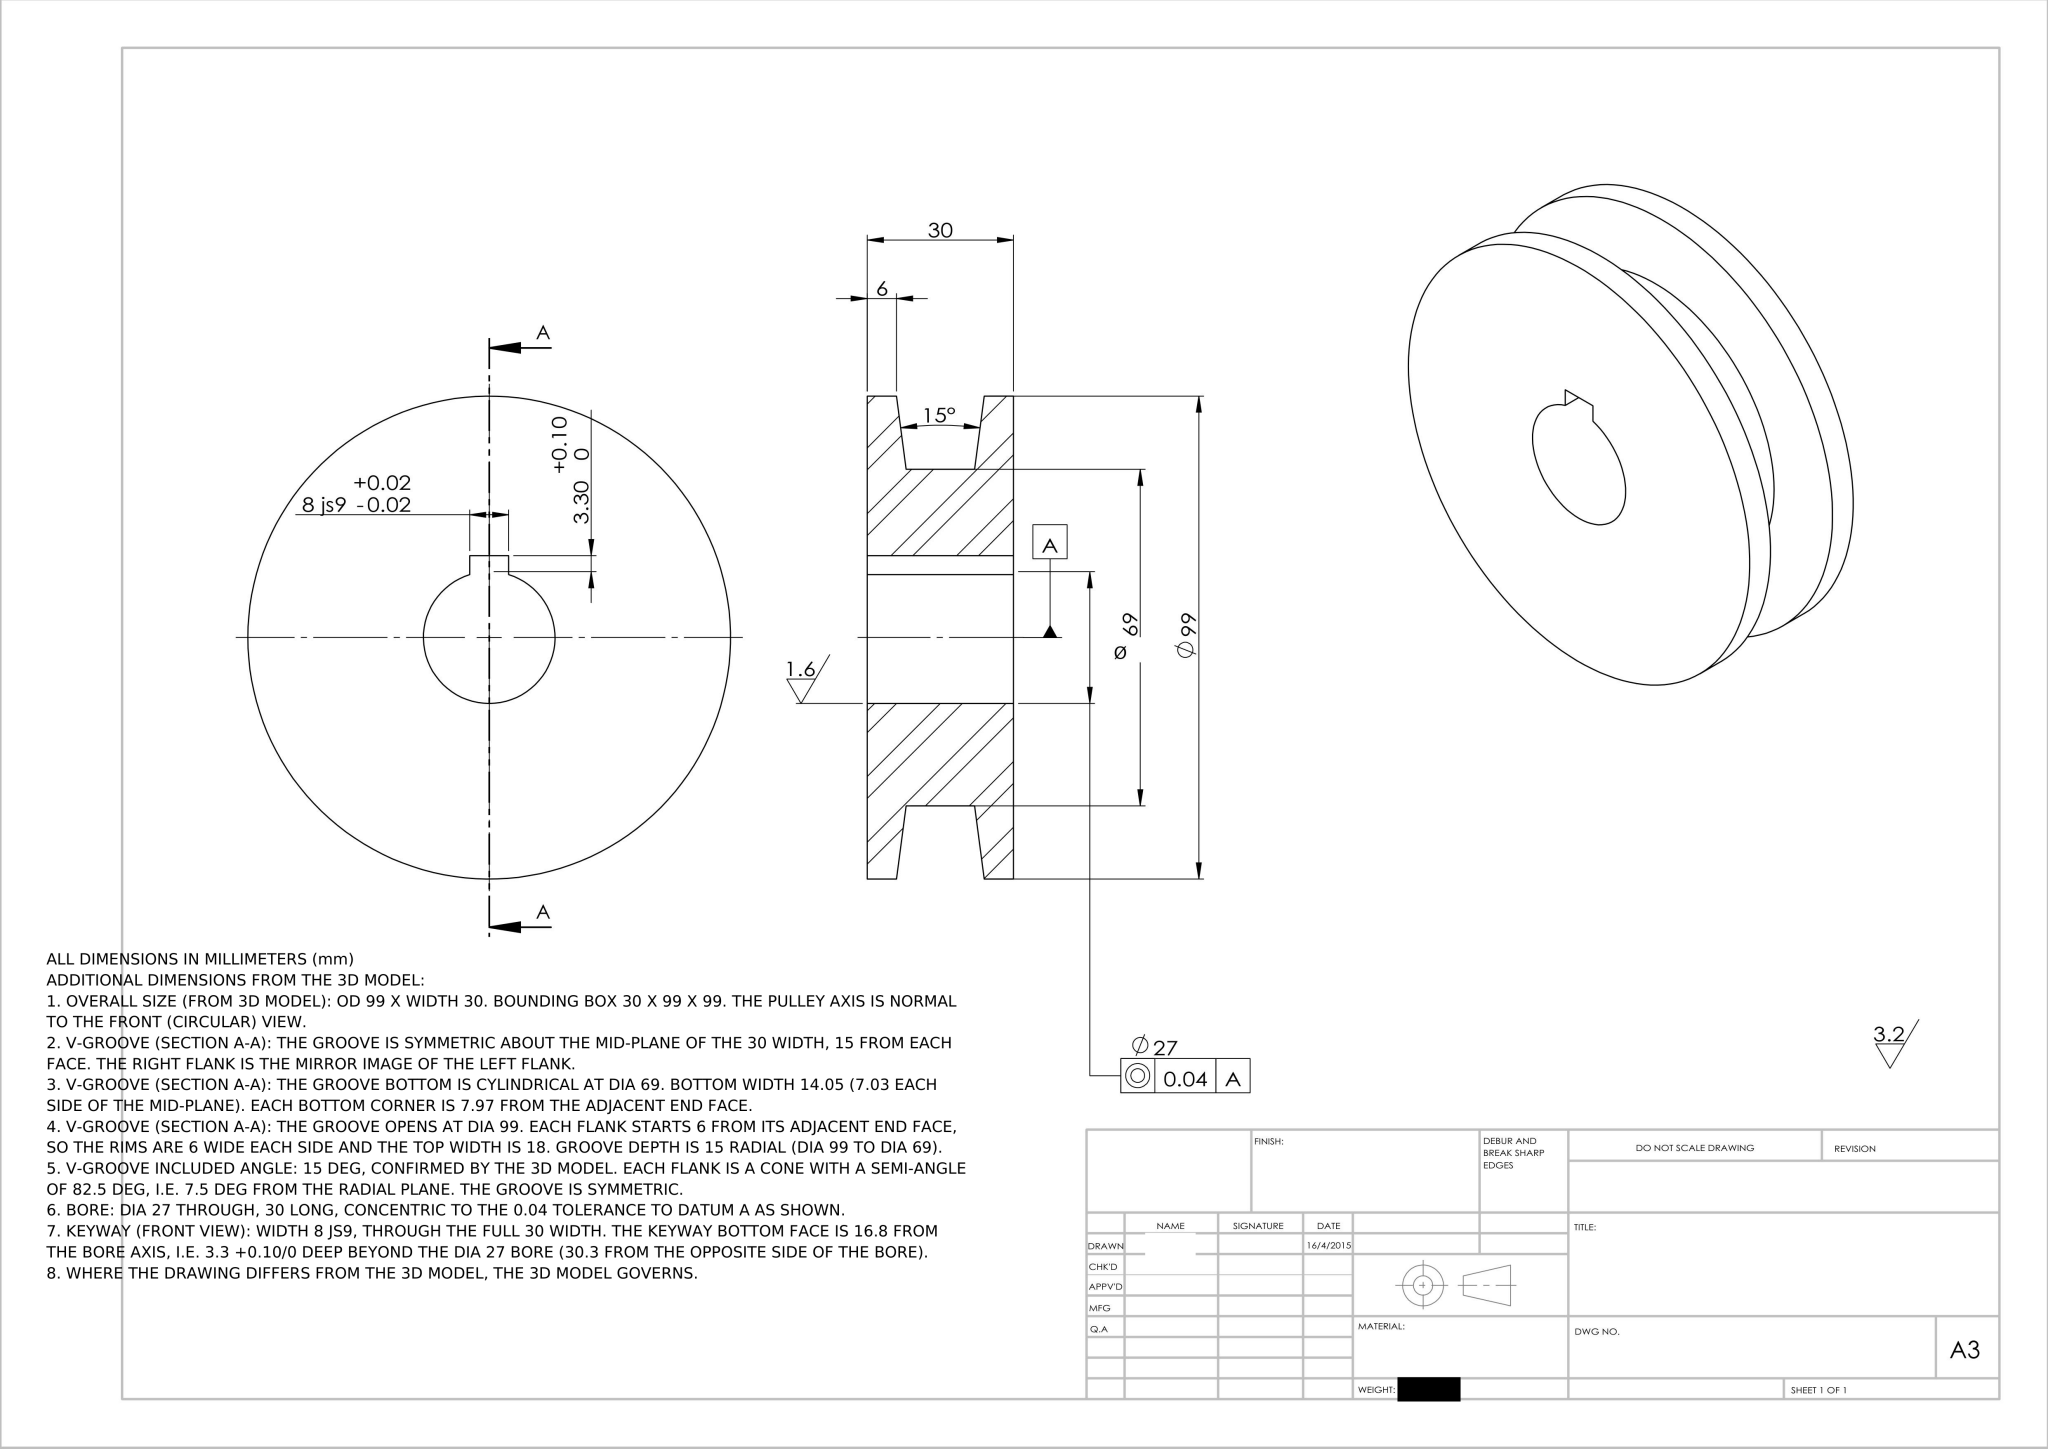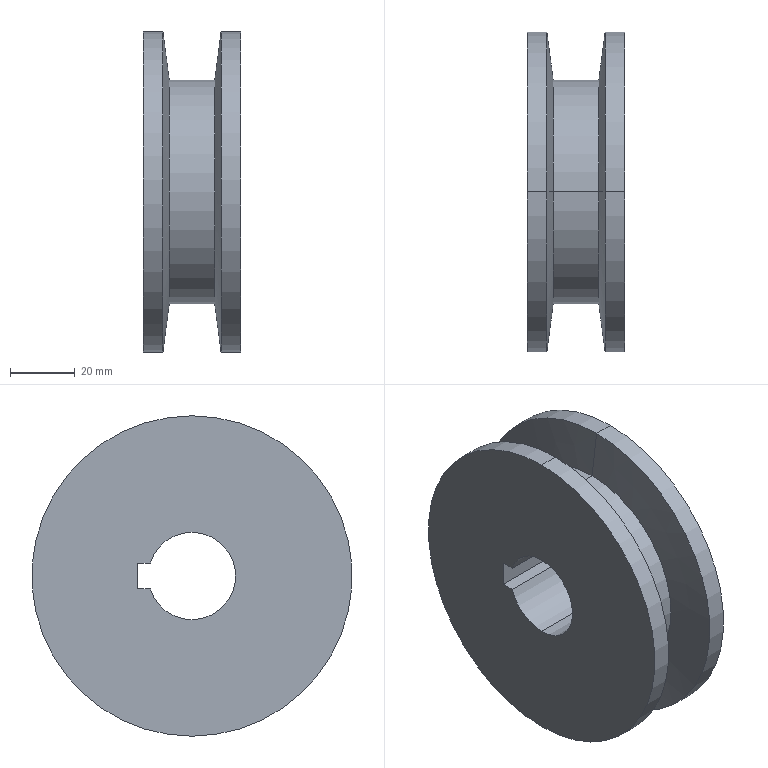Part | NX | mm | Keyed Bore Flanged Pulley | 1 solid | 18 faces | box 30 x 99 x 99 mm | volume 149014 mm3 | cylinder 9 | plane 5 | cone 4 | commonest cylinder face diameters 99 x4 27 x3 69 x2
STEP:
#1=COLOUR_RGB('',0.7922,0.8196,0.9333);
#2=FILL_AREA_STYLE_COLOUR('',#1);
#3=FILL_AREA_STYLE('',(#2));
#4=SURFACE_STYLE_FILL_AREA(#3);
#5=SURFACE_SIDE_STYLE('',(#4));
#6=SURFACE_STYLE_USAGE(.BOTH.,#5);
#7=PRESENTATION_STYLE_ASSIGNMENT((#6));
#8=CARTESIAN_POINT('',(15.,0.,49.5));
#9=VERTEX_POINT('',#8);
#10=CARTESIAN_POINT('',(15.,0.,-49.5));
#11=VERTEX_POINT('',#10);
#12=CARTESIAN_POINT('',(15.,0.,0.));
#13=DIRECTION('',(-1.,0.,0.));
#14=DIRECTION('',(0.,0.,1.));
#15=AXIS2_PLACEMENT_3D('',#12,#13,#14);
#16=CIRCLE('',#15,49.5);
#17=EDGE_CURVE('',#9,#11,#16,.T.);
#18=ORIENTED_EDGE('',*,*,#17,.T.);
#19=CARTESIAN_POINT('',(9.,0.,-49.5));
#20=VERTEX_POINT('',#19);
#21=CARTESIAN_POINT('',(0.,0.,-49.5));
#22=DIRECTION('',(-1.,0.,0.));
#23=VECTOR('',#22,1000.);
#24=LINE('',#21,#23);
#25=EDGE_CURVE('',#11,#20,#24,.T.);
#26=ORIENTED_EDGE('',*,*,#25,.T.);
#27=CARTESIAN_POINT('',(9.,0.,49.5));
#28=VERTEX_POINT('',#27);
#29=CARTESIAN_POINT('',(9.,0.,0.));
#30=DIRECTION('',(-1.,0.,0.));
#31=DIRECTION('',(0.,0.,1.));
#32=AXIS2_PLACEMENT_3D('',#29,#30,#31);
#33=CIRCLE('',#32,49.5);
#34=EDGE_CURVE('',#28,#20,#33,.T.);
#35=ORIENTED_EDGE('',*,*,#34,.F.);
#36=CARTESIAN_POINT('',(0.,0.,49.5));
#37=DIRECTION('',(-1.,0.,0.));
#38=VECTOR('',#37,1000.);
#39=LINE('',#36,#38);
#40=EDGE_CURVE('',#9,#28,#39,.T.);
#41=ORIENTED_EDGE('',*,*,#40,.F.);
#42=EDGE_LOOP('',(#18,#26,#35,#41));
#43=FACE_OUTER_BOUND('',#42,.T.);
#44=CARTESIAN_POINT('',(0.,0.,0.));
#45=DIRECTION('',(-1.,0.,0.));
#46=DIRECTION('',(0.,0.,1.));
#47=AXIS2_PLACEMENT_3D('',#44,#45,#46);
#48=CYLINDRICAL_SURFACE('',#47,49.5);
#49=ADVANCED_FACE('',(#43),#48,.T.);
#50=CARTESIAN_POINT('',(7.025,0.,34.5));
#51=VERTEX_POINT('',#50);
#52=CARTESIAN_POINT('',(7.025,0.,-34.5));
#53=VERTEX_POINT('',#52);
#54=CARTESIAN_POINT('',(7.025,0.,0.));
#55=DIRECTION('',(-1.,0.,0.));
#56=DIRECTION('',(0.,0.,1.));
#57=AXIS2_PLACEMENT_3D('',#54,#55,#56);
#58=CIRCLE('',#57,34.5);
#59=EDGE_CURVE('',#51,#53,#58,.T.);
#60=ORIENTED_EDGE('',*,*,#59,.F.);
#61=CARTESIAN_POINT('',(9.,0.,49.5));
#62=DIRECTION('',(0.1305,0.,0.9914));
#63=VECTOR('',#62,1000.);
#64=LINE('',#61,#63);
#65=EDGE_CURVE('',#51,#28,#64,.T.);
#66=ORIENTED_EDGE('',*,*,#65,.T.);
#67=ORIENTED_EDGE('',*,*,#34,.T.);
#68=CARTESIAN_POINT('',(9.,0.,-49.5));
#69=DIRECTION('',(0.1305,0.,-0.9914));
#70=VECTOR('',#69,1000.);
#71=LINE('',#68,#70);
#72=EDGE_CURVE('',#53,#20,#71,.T.);
#73=ORIENTED_EDGE('',*,*,#72,.F.);
#74=EDGE_LOOP('',(#60,#66,#67,#73));
#75=FACE_OUTER_BOUND('',#74,.T.);
#76=CARTESIAN_POINT('',(9.,0.,0.));
#77=DIRECTION('',(1.,0.,0.));
#78=DIRECTION('',(0.,0.,-1.));
#79=AXIS2_PLACEMENT_3D('',#76,#77,#78);
#80=CONICAL_SURFACE('',#79,49.5,1.44);
#81=ADVANCED_FACE('',(#75),#80,.T.);
#82=ORIENTED_EDGE('',*,*,#59,.T.);
#83=CARTESIAN_POINT('',(-7.025,0.,-34.5));
#84=VERTEX_POINT('',#83);
#85=CARTESIAN_POINT('',(0.,0.,-34.5));
#86=DIRECTION('',(-1.,0.,0.));
#87=VECTOR('',#86,1000.);
#88=LINE('',#85,#87);
#89=EDGE_CURVE('',#53,#84,#88,.T.);
#90=ORIENTED_EDGE('',*,*,#89,.T.);
#91=CARTESIAN_POINT('',(-7.025,0.,34.5));
#92=VERTEX_POINT('',#91);
#93=CARTESIAN_POINT('',(-7.025,0.,0.));
#94=DIRECTION('',(-1.,0.,0.));
#95=DIRECTION('',(0.,0.,1.));
#96=AXIS2_PLACEMENT_3D('',#93,#94,#95);
#97=CIRCLE('',#96,34.5);
#98=EDGE_CURVE('',#92,#84,#97,.T.);
#99=ORIENTED_EDGE('',*,*,#98,.F.);
#100=CARTESIAN_POINT('',(0.,0.,34.5));
#101=DIRECTION('',(-1.,0.,0.));
#102=VECTOR('',#101,1000.);
#103=LINE('',#100,#102);
#104=EDGE_CURVE('',#51,#92,#103,.T.);
#105=ORIENTED_EDGE('',*,*,#104,.F.);
#106=EDGE_LOOP('',(#82,#90,#99,#105));
#107=FACE_OUTER_BOUND('',#106,.T.);
#108=CARTESIAN_POINT('',(0.,0.,0.));
#109=DIRECTION('',(-1.,0.,0.));
#110=DIRECTION('',(0.,0.,1.));
#111=AXIS2_PLACEMENT_3D('',#108,#109,#110);
#112=CYLINDRICAL_SURFACE('',#111,34.5);
#113=ADVANCED_FACE('',(#107),#112,.T.);
#114=ORIENTED_EDGE('',*,*,#98,.T.);
#115=CARTESIAN_POINT('',(-9.,0.,-49.5));
#116=VERTEX_POINT('',#115);
#117=CARTESIAN_POINT('',(-7.025,0.,-34.5));
#118=DIRECTION('',(-0.1305,0.,-0.9914));
#119=VECTOR('',#118,1000.);
#120=LINE('',#117,#119);
#121=EDGE_CURVE('',#84,#116,#120,.T.);
#122=ORIENTED_EDGE('',*,*,#121,.T.);
#123=CARTESIAN_POINT('',(-9.,0.,49.5));
#124=VERTEX_POINT('',#123);
#125=CARTESIAN_POINT('',(-9.,0.,0.));
#126=DIRECTION('',(-1.,0.,0.));
#127=DIRECTION('',(0.,0.,1.));
#128=AXIS2_PLACEMENT_3D('',#125,#126,#127);
#129=CIRCLE('',#128,49.5);
#130=EDGE_CURVE('',#124,#116,#129,.T.);
#131=ORIENTED_EDGE('',*,*,#130,.F.);
#132=CARTESIAN_POINT('',(-7.025,0.,34.5));
#133=DIRECTION('',(-0.1305,0.,0.9914));
#134=VECTOR('',#133,1000.);
#135=LINE('',#132,#134);
#136=EDGE_CURVE('',#92,#124,#135,.T.);
#137=ORIENTED_EDGE('',*,*,#136,.F.);
#138=EDGE_LOOP('',(#114,#122,#131,#137));
#139=FACE_OUTER_BOUND('',#138,.T.);
#140=CARTESIAN_POINT('',(-7.025,0.,0.));
#141=DIRECTION('',(-1.,0.,0.));
#142=DIRECTION('',(0.,0.,1.));
#143=AXIS2_PLACEMENT_3D('',#140,#141,#142);
#144=CONICAL_SURFACE('',#143,34.5,1.44);
#145=ADVANCED_FACE('',(#139),#144,.T.);
#146=ORIENTED_EDGE('',*,*,#130,.T.);
#147=CARTESIAN_POINT('',(-15.,0.,-49.5));
#148=VERTEX_POINT('',#147);
#149=CARTESIAN_POINT('',(0.,0.,-49.5));
#150=DIRECTION('',(-1.,0.,0.));
#151=VECTOR('',#150,1000.);
#152=LINE('',#149,#151);
#153=EDGE_CURVE('',#116,#148,#152,.T.);
#154=ORIENTED_EDGE('',*,*,#153,.T.);
#155=CARTESIAN_POINT('',(-15.,0.,49.5));
#156=VERTEX_POINT('',#155);
#157=CARTESIAN_POINT('',(-15.,0.,0.));
#158=DIRECTION('',(-1.,0.,0.));
#159=DIRECTION('',(0.,0.,1.));
#160=AXIS2_PLACEMENT_3D('',#157,#158,#159);
#161=CIRCLE('',#160,49.5);
#162=EDGE_CURVE('',#156,#148,#161,.T.);
#163=ORIENTED_EDGE('',*,*,#162,.F.);
#164=CARTESIAN_POINT('',(0.,0.,49.5));
#165=DIRECTION('',(-1.,0.,0.));
#166=VECTOR('',#165,1000.);
#167=LINE('',#164,#166);
#168=EDGE_CURVE('',#124,#156,#167,.T.);
#169=ORIENTED_EDGE('',*,*,#168,.F.);
#170=EDGE_LOOP('',(#146,#154,#163,#169));
#171=FACE_OUTER_BOUND('',#170,.T.);
#172=CARTESIAN_POINT('',(0.,0.,0.));
#173=DIRECTION('',(-1.,0.,0.));
#174=DIRECTION('',(0.,0.,1.));
#175=AXIS2_PLACEMENT_3D('',#172,#173,#174);
#176=CYLINDRICAL_SURFACE('',#175,49.5);
#177=ADVANCED_FACE('',(#171),#176,.T.);
#178=CARTESIAN_POINT('',(15.,0.,-13.5));
#179=VERTEX_POINT('',#178);
#180=CARTESIAN_POINT('',(15.,0.,13.5));
#181=VERTEX_POINT('',#180);
#182=CARTESIAN_POINT('',(15.,0.,0.));
#183=DIRECTION('',(-1.,0.,0.));
#184=DIRECTION('',(0.,0.,1.));
#185=AXIS2_PLACEMENT_3D('',#182,#183,#184);
#186=CIRCLE('',#185,13.5);
#187=EDGE_CURVE('',#179,#181,#186,.T.);
#188=ORIENTED_EDGE('',*,*,#187,.F.);
#189=CARTESIAN_POINT('',(-15.,0.,-13.5));
#190=VERTEX_POINT('',#189);
#191=CARTESIAN_POINT('',(0.,0.,-13.5));
#192=DIRECTION('',(-1.,0.,0.));
#193=VECTOR('',#192,1000.);
#194=LINE('',#191,#193);
#195=EDGE_CURVE('',#179,#190,#194,.T.);
#196=ORIENTED_EDGE('',*,*,#195,.T.);
#197=CARTESIAN_POINT('',(-15.,0.,13.5));
#198=VERTEX_POINT('',#197);
#199=CARTESIAN_POINT('',(-15.,0.,0.));
#200=DIRECTION('',(-1.,0.,0.));
#201=DIRECTION('',(0.,0.,1.));
#202=AXIS2_PLACEMENT_3D('',#199,#200,#201);
#203=CIRCLE('',#202,13.5);
#204=EDGE_CURVE('',#190,#198,#203,.T.);
#205=ORIENTED_EDGE('',*,*,#204,.T.);
#206=CARTESIAN_POINT('',(0.,0.,13.5));
#207=DIRECTION('',(-1.,0.,0.));
#208=VECTOR('',#207,1000.);
#209=LINE('',#206,#208);
#210=EDGE_CURVE('',#181,#198,#209,.T.);
#211=ORIENTED_EDGE('',*,*,#210,.F.);
#212=EDGE_LOOP('',(#188,#196,#205,#211));
#213=FACE_OUTER_BOUND('',#212,.T.);
#214=CARTESIAN_POINT('',(0.,0.,0.));
#215=DIRECTION('',(-1.,0.,0.));
#216=DIRECTION('',(0.,0.,1.));
#217=AXIS2_PLACEMENT_3D('',#214,#215,#216);
#218=CYLINDRICAL_SURFACE('',#217,13.5);
#219=ADVANCED_FACE('',(#213),#218,.F.);
#220=CARTESIAN_POINT('',(15.,12.894,4.));
#221=VERTEX_POINT('',#220);
#222=CARTESIAN_POINT('',(15.,0.,0.));
#223=DIRECTION('',(-1.,0.,0.));
#224=DIRECTION('',(0.,0.,1.));
#225=AXIS2_PLACEMENT_3D('',#222,#223,#224);
#226=CIRCLE('',#225,13.5);
#227=EDGE_CURVE('',#181,#221,#226,.T.);
#228=ORIENTED_EDGE('',*,*,#227,.F.);
#229=ORIENTED_EDGE('',*,*,#210,.T.);
#230=CARTESIAN_POINT('',(-15.,12.894,4.));
#231=VERTEX_POINT('',#230);
#232=CARTESIAN_POINT('',(-15.,0.,0.));
#233=DIRECTION('',(-1.,0.,0.));
#234=DIRECTION('',(0.,0.,1.));
#235=AXIS2_PLACEMENT_3D('',#232,#233,#234);
#236=CIRCLE('',#235,13.5);
#237=EDGE_CURVE('',#198,#231,#236,.T.);
#238=ORIENTED_EDGE('',*,*,#237,.T.);
#239=CARTESIAN_POINT('',(-15.,12.894,4.));
#240=DIRECTION('',(1.,0.,0.));
#241=VECTOR('',#240,1000.);
#242=LINE('',#239,#241);
#243=EDGE_CURVE('',#231,#221,#242,.T.);
#244=ORIENTED_EDGE('',*,*,#243,.T.);
#245=EDGE_LOOP('',(#228,#229,#238,#244));
#246=FACE_OUTER_BOUND('',#245,.T.);
#247=CARTESIAN_POINT('',(0.,0.,0.));
#248=DIRECTION('',(-1.,0.,0.));
#249=DIRECTION('',(0.,0.,1.));
#250=AXIS2_PLACEMENT_3D('',#247,#248,#249);
#251=CYLINDRICAL_SURFACE('',#250,13.5);
#252=ADVANCED_FACE('',(#246),#251,.F.);
#253=ORIENTED_EDGE('',*,*,#195,.F.);
#254=CARTESIAN_POINT('',(15.,12.894,-4.));
#255=VERTEX_POINT('',#254);
#256=CARTESIAN_POINT('',(15.,0.,0.));
#257=DIRECTION('',(-1.,0.,0.));
#258=DIRECTION('',(0.,0.,1.));
#259=AXIS2_PLACEMENT_3D('',#256,#257,#258);
#260=CIRCLE('',#259,13.5);
#261=EDGE_CURVE('',#255,#179,#260,.T.);
#262=ORIENTED_EDGE('',*,*,#261,.F.);
#263=CARTESIAN_POINT('',(-15.,12.894,-4.));
#264=VERTEX_POINT('',#263);
#265=CARTESIAN_POINT('',(-15.,12.894,-4.));
#266=DIRECTION('',(1.,0.,0.));
#267=VECTOR('',#266,1000.);
#268=LINE('',#265,#267);
#269=EDGE_CURVE('',#264,#255,#268,.T.);
#270=ORIENTED_EDGE('',*,*,#269,.F.);
#271=CARTESIAN_POINT('',(-15.,0.,0.));
#272=DIRECTION('',(-1.,0.,0.));
#273=DIRECTION('',(0.,0.,1.));
#274=AXIS2_PLACEMENT_3D('',#271,#272,#273);
#275=CIRCLE('',#274,13.5);
#276=EDGE_CURVE('',#264,#190,#275,.T.);
#277=ORIENTED_EDGE('',*,*,#276,.T.);
#278=EDGE_LOOP('',(#253,#262,#270,#277));
#279=FACE_OUTER_BOUND('',#278,.T.);
#280=CARTESIAN_POINT('',(0.,0.,0.));
#281=DIRECTION('',(-1.,0.,0.));
#282=DIRECTION('',(0.,0.,1.));
#283=AXIS2_PLACEMENT_3D('',#280,#281,#282);
#284=CYLINDRICAL_SURFACE('',#283,13.5);
#285=ADVANCED_FACE('',(#279),#284,.F.);
#286=CARTESIAN_POINT('',(-15.,16.8,-4.));
#287=VERTEX_POINT('',#286);
#288=CARTESIAN_POINT('',(-15.,16.8,4.));
#289=VERTEX_POINT('',#288);
#290=CARTESIAN_POINT('',(-15.,16.8,4.));
#291=DIRECTION('',(0.,0.,1.));
#292=VECTOR('',#291,1000.);
#293=LINE('',#290,#292);
#294=EDGE_CURVE('',#287,#289,#293,.T.);
#295=ORIENTED_EDGE('',*,*,#294,.T.);
#296=CARTESIAN_POINT('',(-15.,12.894,4.));
#297=DIRECTION('',(0.,-1.,0.));
#298=VECTOR('',#297,1000.);
#299=LINE('',#296,#298);
#300=EDGE_CURVE('',#289,#231,#299,.T.);
#301=ORIENTED_EDGE('',*,*,#300,.T.);
#302=ORIENTED_EDGE('',*,*,#237,.F.);
#303=ORIENTED_EDGE('',*,*,#204,.F.);
#304=ORIENTED_EDGE('',*,*,#276,.F.);
#305=CARTESIAN_POINT('',(-15.,16.8,-4.));
#306=DIRECTION('',(0.,1.,0.));
#307=VECTOR('',#306,1000.);
#308=LINE('',#305,#307);
#309=EDGE_CURVE('',#264,#287,#308,.T.);
#310=ORIENTED_EDGE('',*,*,#309,.T.);
#311=EDGE_LOOP('',(#295,#301,#302,#303,#304,#310));
#312=FACE_BOUND('',#311,.T.);
#313=ORIENTED_EDGE('',*,*,#162,.T.);
#314=CARTESIAN_POINT('',(-15.,0.,0.));
#315=DIRECTION('',(-1.,0.,0.));
#316=DIRECTION('',(0.,0.,1.));
#317=AXIS2_PLACEMENT_3D('',#314,#315,#316);
#318=CIRCLE('',#317,49.5);
#319=EDGE_CURVE('',#148,#156,#318,.T.);
#320=ORIENTED_EDGE('',*,*,#319,.T.);
#321=EDGE_LOOP('',(#313,#320));
#322=FACE_OUTER_BOUND('',#321,.T.);
#323=CARTESIAN_POINT('',(-15.,13.5,0.));
#324=DIRECTION('',(1.,0.,0.));
#325=DIRECTION('',(0.,0.,-1.));
#326=AXIS2_PLACEMENT_3D('',#323,#324,#325);
#327=PLANE('',#326);
#328=ADVANCED_FACE('',(#312,#322),#327,.F.);
#329=ORIENTED_EDGE('',*,*,#153,.F.);
#330=CARTESIAN_POINT('',(-9.,0.,0.));
#331=DIRECTION('',(-1.,0.,0.));
#332=DIRECTION('',(0.,0.,1.));
#333=AXIS2_PLACEMENT_3D('',#330,#331,#332);
#334=CIRCLE('',#333,49.5);
#335=EDGE_CURVE('',#116,#124,#334,.T.);
#336=ORIENTED_EDGE('',*,*,#335,.T.);
#337=ORIENTED_EDGE('',*,*,#168,.T.);
#338=ORIENTED_EDGE('',*,*,#319,.F.);
#339=EDGE_LOOP('',(#329,#336,#337,#338));
#340=FACE_OUTER_BOUND('',#339,.T.);
#341=CARTESIAN_POINT('',(0.,0.,0.));
#342=DIRECTION('',(-1.,0.,0.));
#343=DIRECTION('',(0.,0.,1.));
#344=AXIS2_PLACEMENT_3D('',#341,#342,#343);
#345=CYLINDRICAL_SURFACE('',#344,49.5);
#346=ADVANCED_FACE('',(#340),#345,.T.);
#347=ORIENTED_EDGE('',*,*,#121,.F.);
#348=CARTESIAN_POINT('',(-7.025,0.,0.));
#349=DIRECTION('',(-1.,0.,0.));
#350=DIRECTION('',(0.,0.,1.));
#351=AXIS2_PLACEMENT_3D('',#348,#349,#350);
#352=CIRCLE('',#351,34.5);
#353=EDGE_CURVE('',#84,#92,#352,.T.);
#354=ORIENTED_EDGE('',*,*,#353,.T.);
#355=ORIENTED_EDGE('',*,*,#136,.T.);
#356=ORIENTED_EDGE('',*,*,#335,.F.);
#357=EDGE_LOOP('',(#347,#354,#355,#356));
#358=FACE_OUTER_BOUND('',#357,.T.);
#359=CARTESIAN_POINT('',(-7.025,0.,0.));
#360=DIRECTION('',(-1.,0.,0.));
#361=DIRECTION('',(0.,0.,1.));
#362=AXIS2_PLACEMENT_3D('',#359,#360,#361);
#363=CONICAL_SURFACE('',#362,34.5,1.44);
#364=ADVANCED_FACE('',(#358),#363,.T.);
#365=ORIENTED_EDGE('',*,*,#89,.F.);
#366=CARTESIAN_POINT('',(7.025,0.,0.));
#367=DIRECTION('',(-1.,0.,0.));
#368=DIRECTION('',(0.,0.,1.));
#369=AXIS2_PLACEMENT_3D('',#366,#367,#368);
#370=CIRCLE('',#369,34.5);
#371=EDGE_CURVE('',#53,#51,#370,.T.);
#372=ORIENTED_EDGE('',*,*,#371,.T.);
#373=ORIENTED_EDGE('',*,*,#104,.T.);
#374=ORIENTED_EDGE('',*,*,#353,.F.);
#375=EDGE_LOOP('',(#365,#372,#373,#374));
#376=FACE_OUTER_BOUND('',#375,.T.);
#377=CARTESIAN_POINT('',(0.,0.,0.));
#378=DIRECTION('',(-1.,0.,0.));
#379=DIRECTION('',(0.,0.,1.));
#380=AXIS2_PLACEMENT_3D('',#377,#378,#379);
#381=CYLINDRICAL_SURFACE('',#380,34.5);
#382=ADVANCED_FACE('',(#376),#381,.T.);
#383=ORIENTED_EDGE('',*,*,#65,.F.);
#384=ORIENTED_EDGE('',*,*,#371,.F.);
#385=ORIENTED_EDGE('',*,*,#72,.T.);
#386=CARTESIAN_POINT('',(9.,0.,0.));
#387=DIRECTION('',(-1.,0.,0.));
#388=DIRECTION('',(0.,0.,1.));
#389=AXIS2_PLACEMENT_3D('',#386,#387,#388);
#390=CIRCLE('',#389,49.5);
#391=EDGE_CURVE('',#20,#28,#390,.T.);
#392=ORIENTED_EDGE('',*,*,#391,.T.);
#393=EDGE_LOOP('',(#383,#384,#385,#392));
#394=FACE_OUTER_BOUND('',#393,.T.);
#395=CARTESIAN_POINT('',(9.,0.,0.));
#396=DIRECTION('',(1.,0.,0.));
#397=DIRECTION('',(0.,0.,-1.));
#398=AXIS2_PLACEMENT_3D('',#395,#396,#397);
#399=CONICAL_SURFACE('',#398,49.5,1.44);
#400=ADVANCED_FACE('',(#394),#399,.T.);
#401=ORIENTED_EDGE('',*,*,#25,.F.);
#402=CARTESIAN_POINT('',(15.,0.,0.));
#403=DIRECTION('',(-1.,0.,0.));
#404=DIRECTION('',(0.,0.,1.));
#405=AXIS2_PLACEMENT_3D('',#402,#403,#404);
#406=CIRCLE('',#405,49.5);
#407=EDGE_CURVE('',#11,#9,#406,.T.);
#408=ORIENTED_EDGE('',*,*,#407,.T.);
#409=ORIENTED_EDGE('',*,*,#40,.T.);
#410=ORIENTED_EDGE('',*,*,#391,.F.);
#411=EDGE_LOOP('',(#401,#408,#409,#410));
#412=FACE_OUTER_BOUND('',#411,.T.);
#413=CARTESIAN_POINT('',(0.,0.,0.));
#414=DIRECTION('',(-1.,0.,0.));
#415=DIRECTION('',(0.,0.,1.));
#416=AXIS2_PLACEMENT_3D('',#413,#414,#415);
#417=CYLINDRICAL_SURFACE('',#416,49.5);
#418=ADVANCED_FACE('',(#412),#417,.T.);
#419=ORIENTED_EDGE('',*,*,#17,.F.);
#420=ORIENTED_EDGE('',*,*,#407,.F.);
#421=EDGE_LOOP('',(#419,#420));
#422=FACE_OUTER_BOUND('',#421,.T.);
#423=ORIENTED_EDGE('',*,*,#261,.T.);
#424=ORIENTED_EDGE('',*,*,#187,.T.);
#425=ORIENTED_EDGE('',*,*,#227,.T.);
#426=CARTESIAN_POINT('',(15.,16.8,4.));
#427=VERTEX_POINT('',#426);
#428=CARTESIAN_POINT('',(15.,12.894,4.));
#429=DIRECTION('',(0.,-1.,0.));
#430=VECTOR('',#429,1000.);
#431=LINE('',#428,#430);
#432=EDGE_CURVE('',#427,#221,#431,.T.);
#433=ORIENTED_EDGE('',*,*,#432,.F.);
#434=CARTESIAN_POINT('',(15.,16.8,-4.));
#435=VERTEX_POINT('',#434);
#436=CARTESIAN_POINT('',(15.,16.8,4.));
#437=DIRECTION('',(0.,0.,1.));
#438=VECTOR('',#437,1000.);
#439=LINE('',#436,#438);
#440=EDGE_CURVE('',#435,#427,#439,.T.);
#441=ORIENTED_EDGE('',*,*,#440,.F.);
#442=CARTESIAN_POINT('',(15.,16.8,-4.));
#443=DIRECTION('',(0.,1.,0.));
#444=VECTOR('',#443,1000.);
#445=LINE('',#442,#444);
#446=EDGE_CURVE('',#255,#435,#445,.T.);
#447=ORIENTED_EDGE('',*,*,#446,.F.);
#448=EDGE_LOOP('',(#423,#424,#425,#433,#441,#447));
#449=FACE_BOUND('',#448,.T.);
#450=CARTESIAN_POINT('',(15.,49.5,0.));
#451=DIRECTION('',(-1.,0.,0.));
#452=DIRECTION('',(0.,0.,1.));
#453=AXIS2_PLACEMENT_3D('',#450,#451,#452);
#454=PLANE('',#453);
#455=ADVANCED_FACE('',(#422,#449),#454,.F.);
#456=ORIENTED_EDGE('',*,*,#432,.T.);
#457=ORIENTED_EDGE('',*,*,#243,.F.);
#458=ORIENTED_EDGE('',*,*,#300,.F.);
#459=CARTESIAN_POINT('',(-15.,16.8,4.));
#460=DIRECTION('',(1.,0.,0.));
#461=VECTOR('',#460,1000.);
#462=LINE('',#459,#461);
#463=EDGE_CURVE('',#289,#427,#462,.T.);
#464=ORIENTED_EDGE('',*,*,#463,.T.);
#465=EDGE_LOOP('',(#456,#457,#458,#464));
#466=FACE_OUTER_BOUND('',#465,.T.);
#467=CARTESIAN_POINT('',(-15.,12.894,4.));
#468=DIRECTION('',(0.,0.,1.));
#469=DIRECTION('',(1.,0.,0.));
#470=AXIS2_PLACEMENT_3D('',#467,#468,#469);
#471=PLANE('',#470);
#472=ADVANCED_FACE('',(#466),#471,.F.);
#473=ORIENTED_EDGE('',*,*,#440,.T.);
#474=ORIENTED_EDGE('',*,*,#463,.F.);
#475=ORIENTED_EDGE('',*,*,#294,.F.);
#476=CARTESIAN_POINT('',(-15.,16.8,-4.));
#477=DIRECTION('',(1.,0.,0.));
#478=VECTOR('',#477,1000.);
#479=LINE('',#476,#478);
#480=EDGE_CURVE('',#287,#435,#479,.T.);
#481=ORIENTED_EDGE('',*,*,#480,.T.);
#482=EDGE_LOOP('',(#473,#474,#475,#481));
#483=FACE_OUTER_BOUND('',#482,.T.);
#484=CARTESIAN_POINT('',(-15.,16.8,4.));
#485=DIRECTION('',(0.,1.,0.));
#486=DIRECTION('',(0.,0.,1.));
#487=AXIS2_PLACEMENT_3D('',#484,#485,#486);
#488=PLANE('',#487);
#489=ADVANCED_FACE('',(#483),#488,.F.);
#490=ORIENTED_EDGE('',*,*,#446,.T.);
#491=ORIENTED_EDGE('',*,*,#480,.F.);
#492=ORIENTED_EDGE('',*,*,#309,.F.);
#493=ORIENTED_EDGE('',*,*,#269,.T.);
#494=EDGE_LOOP('',(#490,#491,#492,#493));
#495=FACE_OUTER_BOUND('',#494,.T.);
#496=CARTESIAN_POINT('',(-15.,16.8,-4.));
#497=DIRECTION('',(0.,0.,-1.));
#498=DIRECTION('',(-1.,0.,0.));
#499=AXIS2_PLACEMENT_3D('',#496,#497,#498);
#500=PLANE('',#499);
#501=ADVANCED_FACE('',(#495),#500,.F.);
#502=CLOSED_SHELL('',(#49,#81,#113,#145,#177,#219,#252,#285,#328,#346,#364,#382,#400,#418,#455,#472,#489,#501));
#503=MANIFOLD_SOLID_BREP('',#502);
#504=STYLED_ITEM('',(#7),#503);
#505=PRESENTATION_LAYER_ASSIGNMENT('','',(#504));
#506=(LENGTH_UNIT()NAMED_UNIT(*)SI_UNIT(.MILLI.,.METRE.));
#507=UNCERTAINTY_MEASURE_WITH_UNIT(LENGTH_MEASURE(0.00001),#506,'','');
#508=(NAMED_UNIT(*)PLANE_ANGLE_UNIT()SI_UNIT($,.RADIAN.));
#509=(NAMED_UNIT(*)SI_UNIT($,.STERADIAN.)SOLID_ANGLE_UNIT());
#510=(GEOMETRIC_REPRESENTATION_CONTEXT(3)GLOBAL_UNCERTAINTY_ASSIGNED_CONTEXT((#507))GLOBAL_UNIT_ASSIGNED_CONTEXT((#506,#508,#509))REPRESENTATION_CONTEXT('',''));
#511=MECHANICAL_DESIGN_GEOMETRIC_PRESENTATION_REPRESENTATION('',(#504),#510);
#512=CARTESIAN_POINT('',(0.,0.,0.));
#513=DIRECTION('',(0.,0.,1.));
#514=DIRECTION('',(1.,0.,0.));
#515=AXIS2_PLACEMENT_3D('',#512,#513,#514);
#516=(LENGTH_UNIT()NAMED_UNIT(*)SI_UNIT(.MILLI.,.METRE.));
#517=UNCERTAINTY_MEASURE_WITH_UNIT(LENGTH_MEASURE(0.00001),#516,'','');
#518=(NAMED_UNIT(*)PLANE_ANGLE_UNIT()SI_UNIT($,.RADIAN.));
#519=(NAMED_UNIT(*)SI_UNIT($,.STERADIAN.)SOLID_ANGLE_UNIT());
#520=(GEOMETRIC_REPRESENTATION_CONTEXT(3)GLOBAL_UNCERTAINTY_ASSIGNED_CONTEXT((#517))GLOBAL_UNIT_ASSIGNED_CONTEXT((#516,#518,#519))REPRESENTATION_CONTEXT('',''));
#521=ADVANCED_BREP_SHAPE_REPRESENTATION('',(#503,#515),#520);